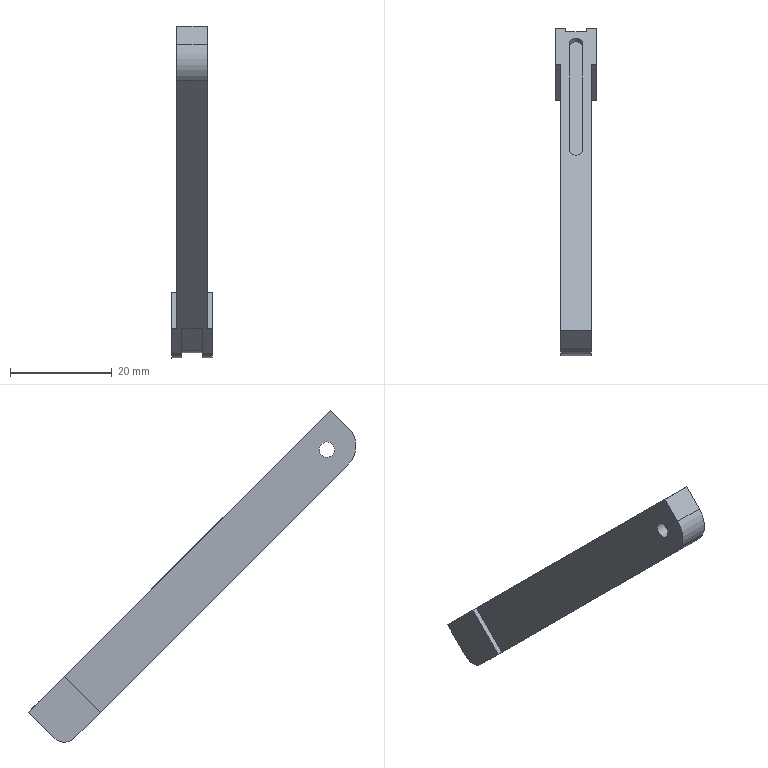Component | SolidWorks | ZL3-10-09PressureBlock-1 | 1 solid | 27 faces | volume 4998 mm3 | plane 19 | cylinder 8 | commonest cylinder face diameters 3 x2 6 x2 2.5 x2 10 x1 4 x1